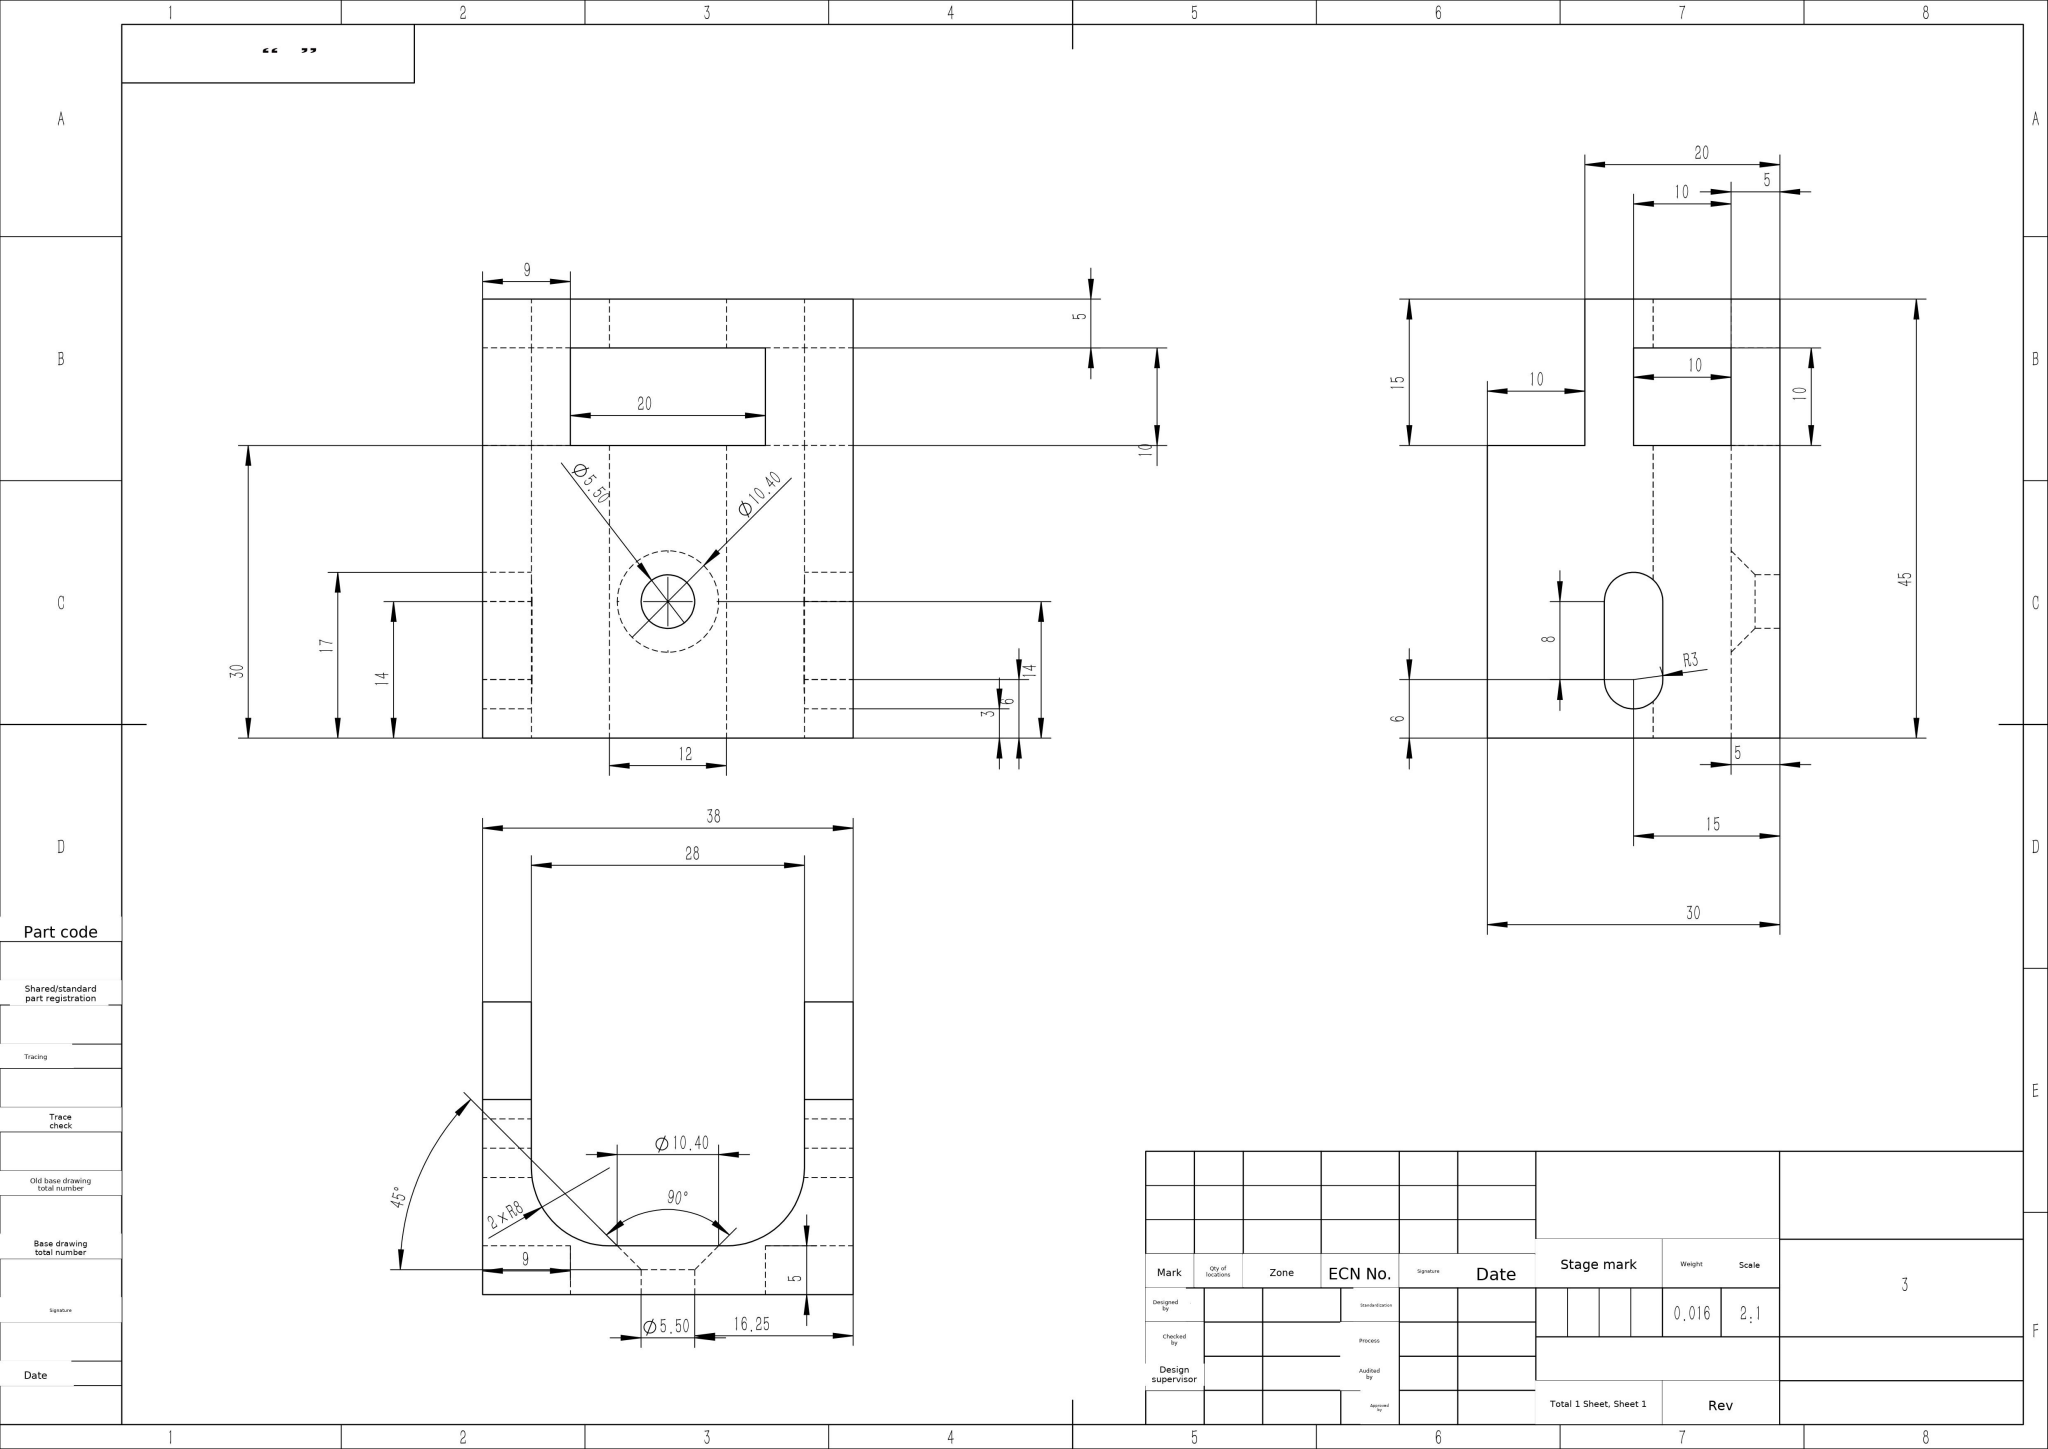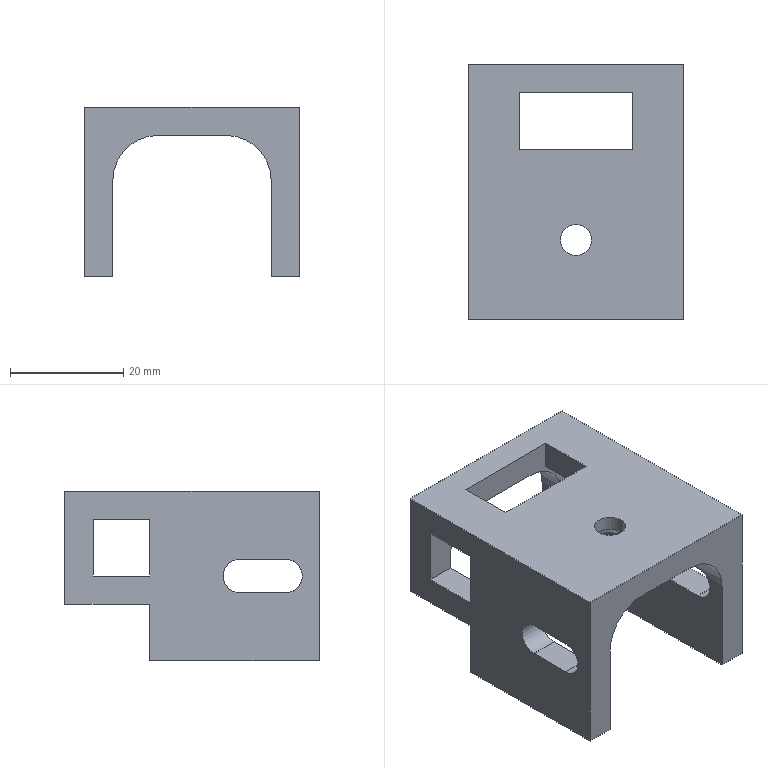Part | SolidWorks | mm | 1 solid | 39 faces | box 38 x 45 x 30 mm | volume 16312 mm3 | plane 27 | cylinder 10 | cone 2 | commonest cylinder face diameters 16 x4 6 x4 5.5 x2
build123d program:
from build123d import *

# Parameters (mm, degrees)
BOSS_EXTRUDE1_DEPTH = 45
FILLET2_R           = 8
SKETCH2_W           = 14.707
SKETCH2_H           = 21.743
SKETCH2_W_2         = 10
SKETCH2_H_2         = 10
CUT_EXTRUDE1_DEPTH  = 50
SKETCH3_W           = 20
SKETCH3_H           = 10
CUT_EXTRUDE2_DEPTH  = 50
HOLE1_D             = 5.5
HOLE1_DEPTH         = 100
HOLE1_CSINK_D       = 10.4
HOLE1_CSINK_ANGLE   = 90
CUT_EXTRUDE3_DEPTH  = 50


with BuildPart() as part:
    # Sketch1 → Boss-Extrude1 (new body)
    with BuildSketch(Plane(origin=(0, 0, 0), x_dir=(1, 0, 0), z_dir=(0, 1, 0))):
        Polygon((-19, 0), (19, 0), (19, 30), (14, 30), (14, 5), (-14, 5), (-14, 30), (-19, 30), align=None)
    extrude(amount=BOSS_EXTRUDE1_DEPTH)

    # Fillet2
    fillet2_edges = [part.edges().sort_by_distance(p)[0] for p in [
        (-14, 22.5, -5),
        (14, 22.5, -5),
    ]]
    fillet(fillet2_edges, radius=FILLET2_R)

    # Sketch2 → Cut-Extrude1 (cut, symmetric)
    with BuildSketch(Plane(origin=(0, 0, 0), x_dir=(0, 0, -1), z_dir=(1, 0, 0))):
        with Locations((27.353, 40.871)):
            Rectangle(SKETCH2_W, SKETCH2_H)
        with Locations((10, 35)):
            Rectangle(SKETCH2_W_2, SKETCH2_H_2)
    extrude(amount=CUT_EXTRUDE1_DEPTH, both=True, mode=Mode.SUBTRACT)

    # Sketch3 → Cut-Extrude2 (cut, symmetric)
    with BuildSketch(Plane.XY):
        with Locations((0, 35)):
            Rectangle(SKETCH3_W, SKETCH3_H)
    extrude(amount=CUT_EXTRUDE2_DEPTH, both=True, mode=Mode.SUBTRACT)

    # Hole1
    with Locations(Plane(origin=(0, 0, -5), x_dir=(-1, 0, 0), z_dir=(0, 0, -1))):
        with Locations((0, 14)):
            CounterSinkHole(HOLE1_D / 2, HOLE1_CSINK_D / 2, depth=HOLE1_DEPTH, counter_sink_angle=HOLE1_CSINK_ANGLE)

    # Sketch8 → Cut-Extrude3 (cut, symmetric)
    with BuildSketch(Plane(origin=(0, 0, 0), x_dir=(0, 0, -1), z_dir=(1, 0, 0))):
        with BuildLine():
            Line((18, 14), (18, 6))
            ThreePointArc((18, 6), (15, 3), (12, 6))
            Line((12, 6), (12, 14))
            ThreePointArc((12, 14), (15, 17), (18, 14))
        make_face()
    extrude(amount=CUT_EXTRUDE3_DEPTH, both=True, mode=Mode.SUBTRACT)


solid = part.part